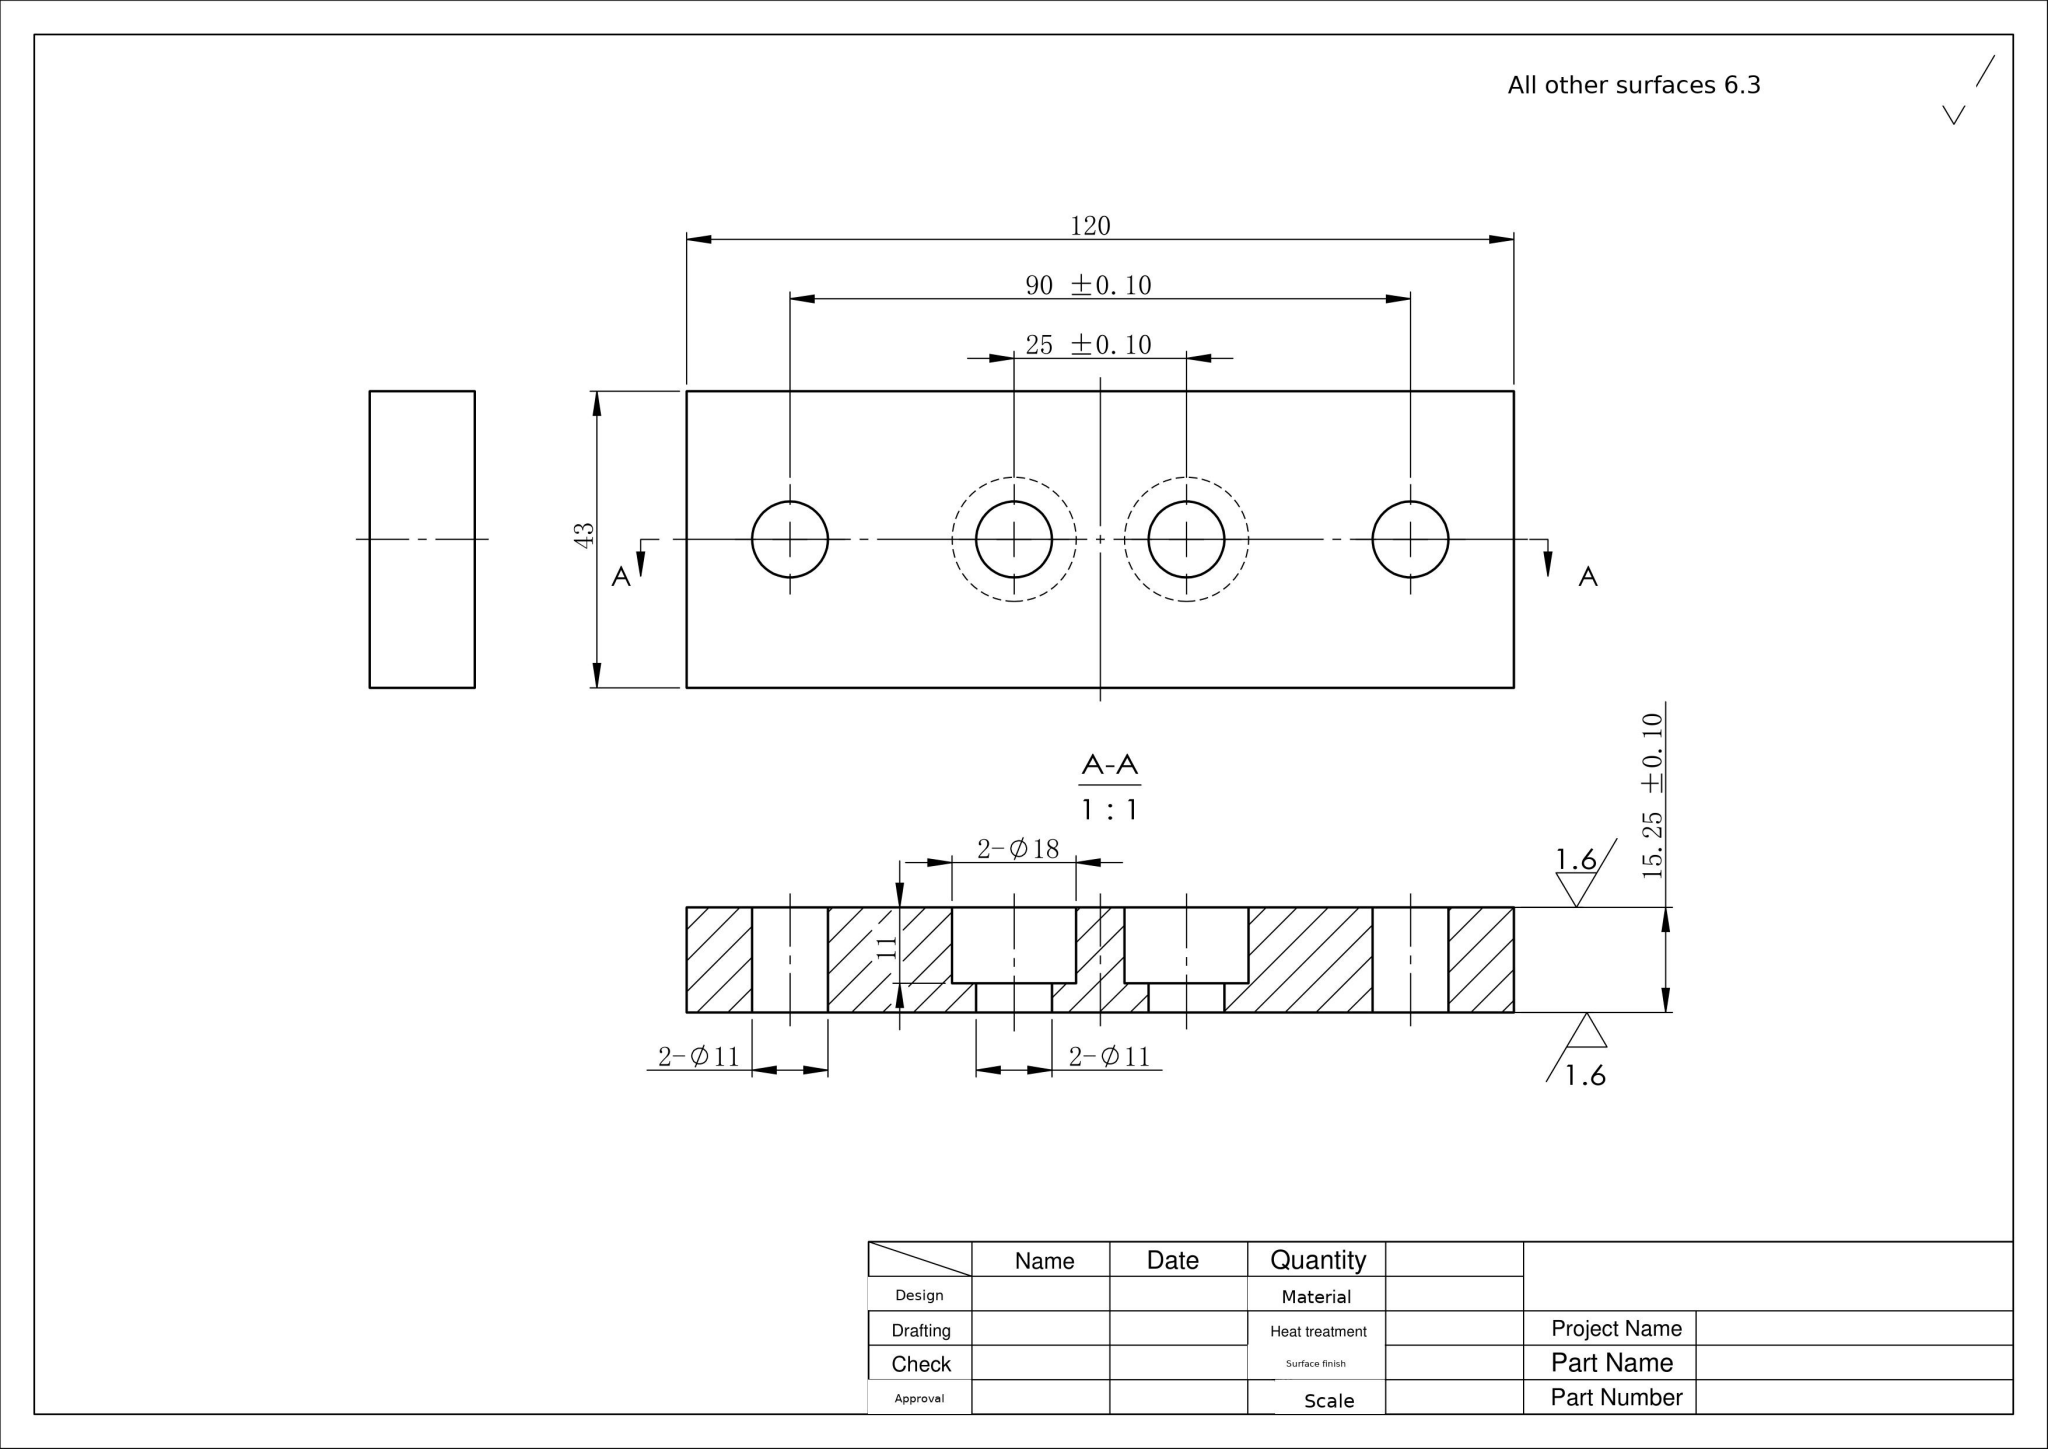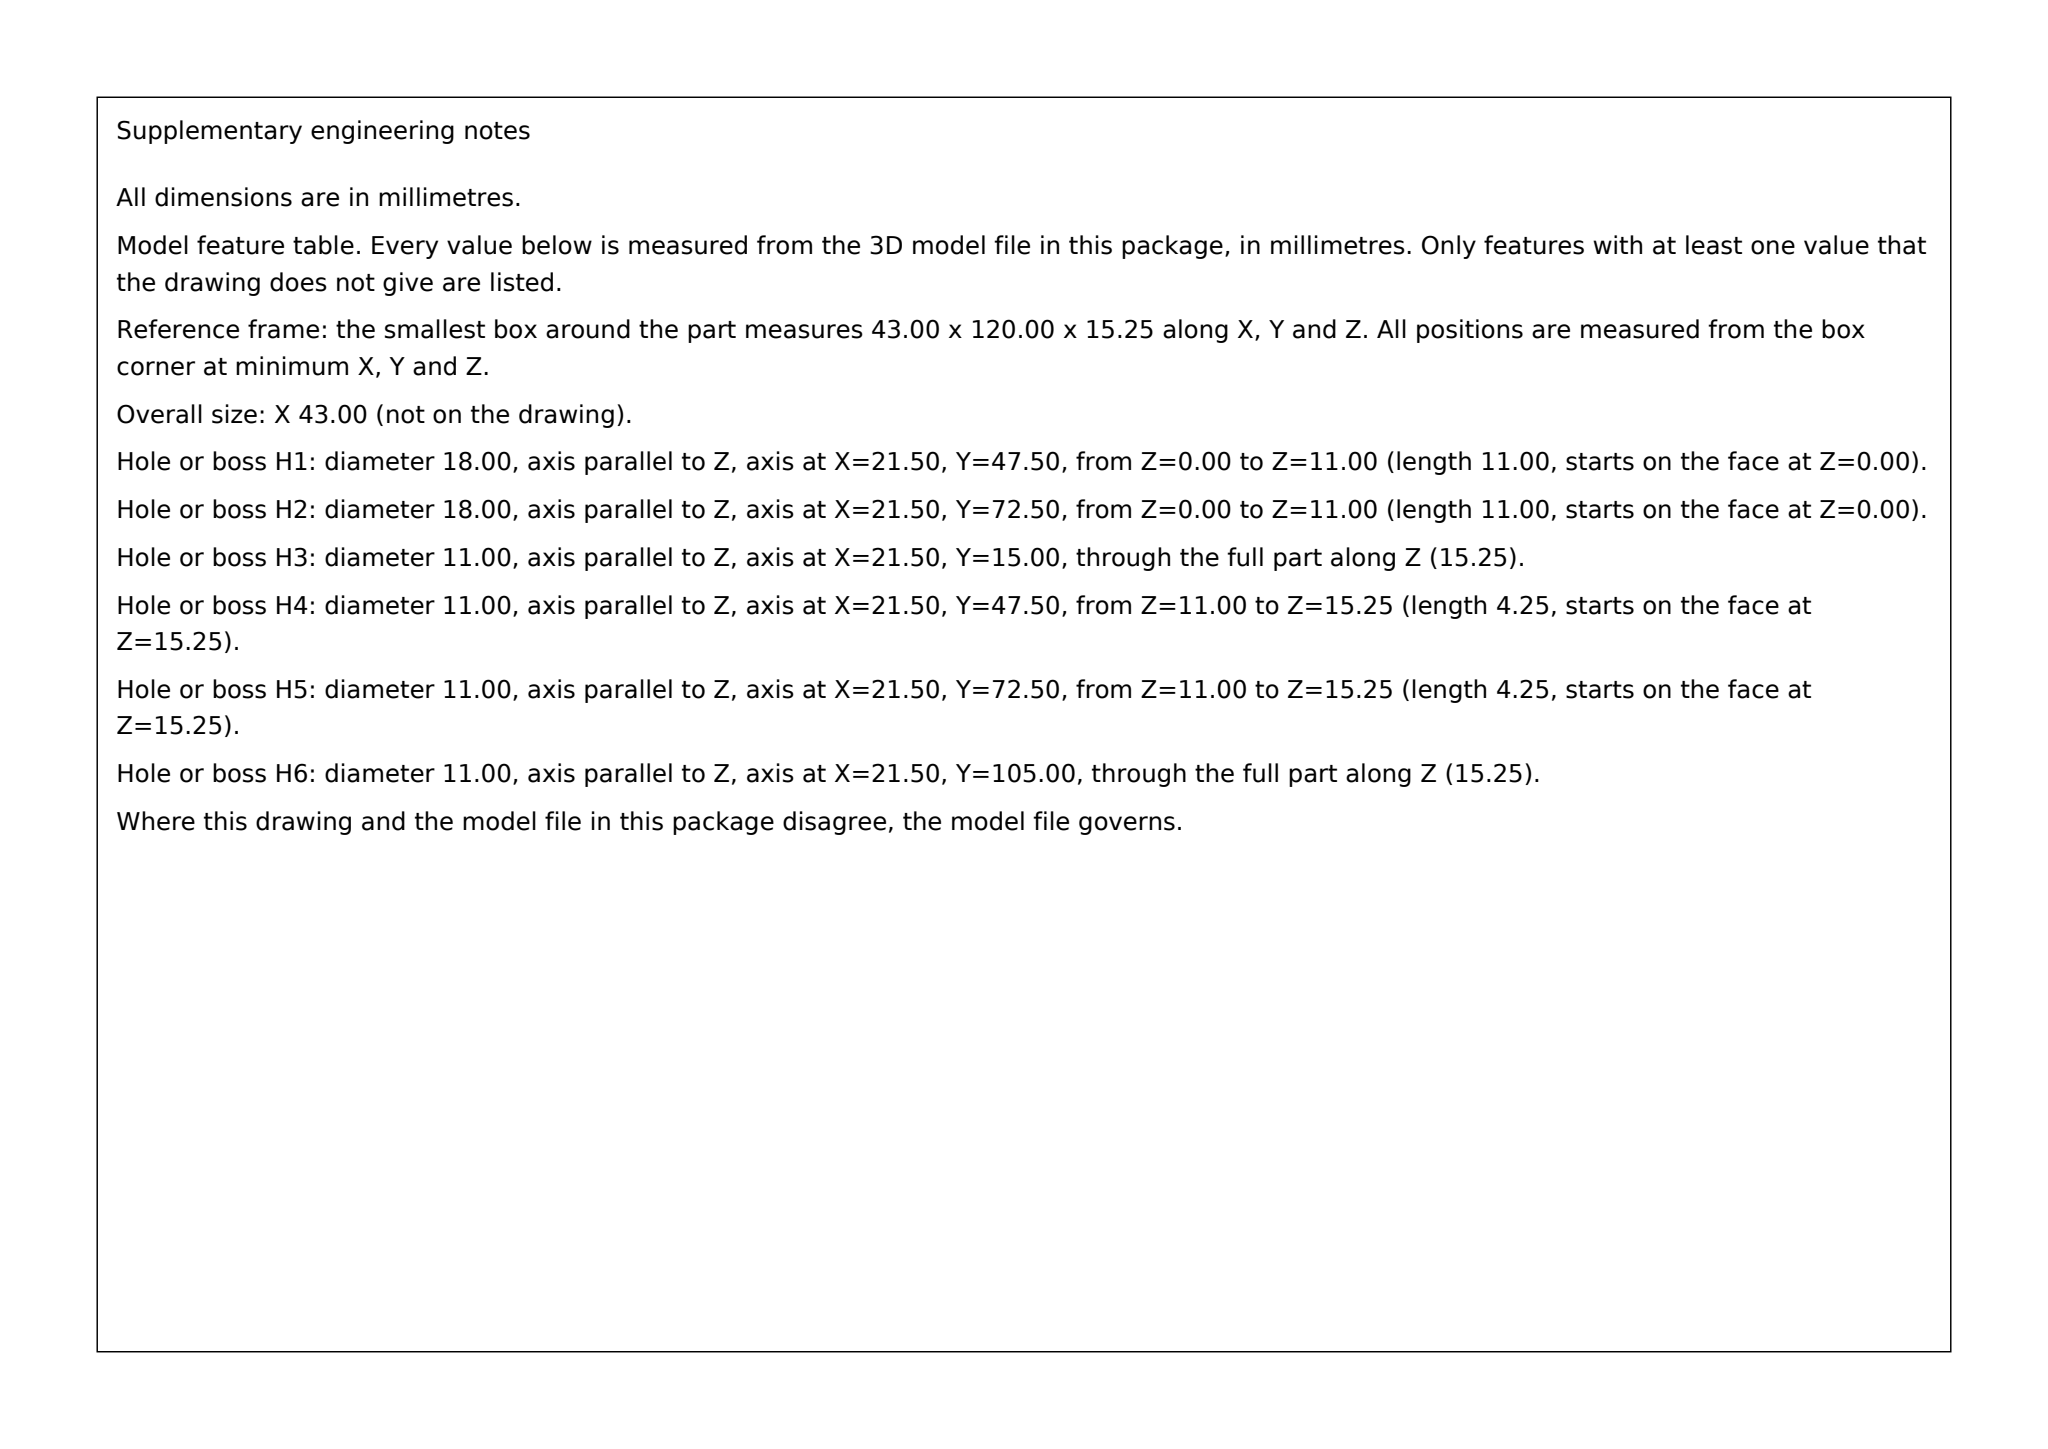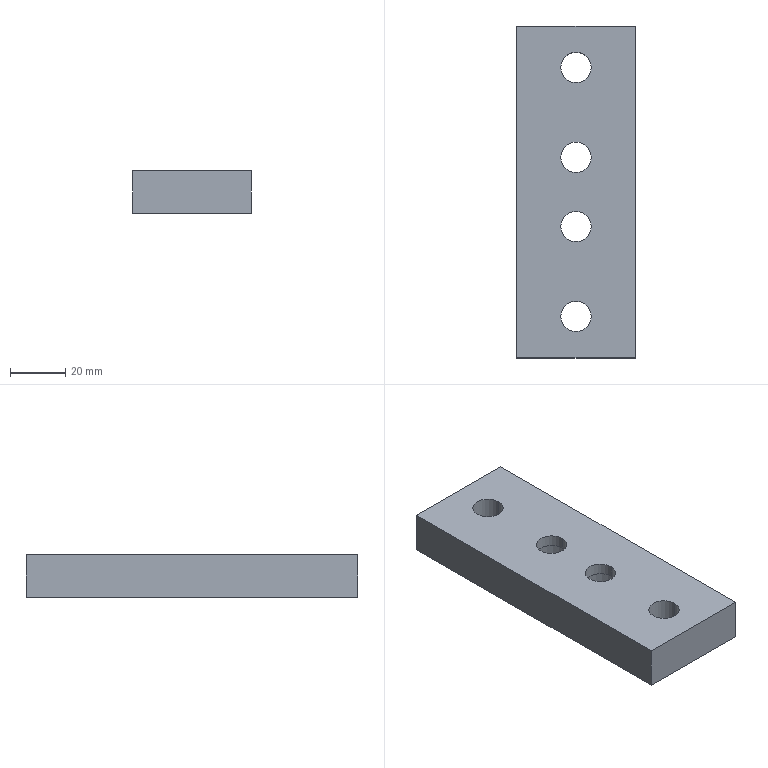Part | SolidWorks | mm | 1 solid | 20 faces | box 43 x 120 x 15.25 mm | volume 69385 mm3 | cylinder 12 | plane 8 | commonest cylinder face diameters 11 x8 18 x4
build123d program:
from build123d import *

# Parameters (mm, degrees)
SKETCH1_W                                        = 43
SKETCH1_H                                        = 120
EXTRUDE1_DEPTH                                   = 15.25
M10_HEX_SOCKET_HEAD_CAP_SCREW_CBORE1_D           = 11
M10_HEX_SOCKET_HEAD_CAP_SCREW_CBORE1_CBORE_D     = 18
M10_HEX_SOCKET_HEAD_CAP_SCREW_CBORE1_CBORE_DEPTH = 11
SKETCH4_R                                        = 5.5
CUT_EXTRUDE1_DEPTH                               = 129.381


with BuildPart() as part:
    # Sketch1 → Extrude1 (new body)
    with BuildSketch(Plane.XY):
        with Locations((21.5, 60)):
            Rectangle(SKETCH1_W, SKETCH1_H)
    extrude(amount=EXTRUDE1_DEPTH)

    # M10 Hex Socket Head Cap Screw CBORE1 (through all)
    with Locations(Plane(origin=(0, 0, 0), x_dir=(-1, 0, 0), z_dir=(0, 0, -1))):
        with Locations((-21.5, 47.5), (-21.5, 72.5)):
            CounterBoreHole(M10_HEX_SOCKET_HEAD_CAP_SCREW_CBORE1_D / 2, M10_HEX_SOCKET_HEAD_CAP_SCREW_CBORE1_CBORE_D / 2, M10_HEX_SOCKET_HEAD_CAP_SCREW_CBORE1_CBORE_DEPTH)

    # Sketch4 → Cut-Extrude1 (cut, through all)
    with BuildSketch(Plane.XY.offset(15.25)):
        with Locations((21.5, 105)):
            Circle(SKETCH4_R)
        with Locations((21.5, 15)):
            Circle(SKETCH4_R)
    extrude(amount=-CUT_EXTRUDE1_DEPTH, mode=Mode.SUBTRACT)


solid = part.part
STEP:
#1=CARTESIAN_POINT('',(16.,15.,0.));
#2=VERTEX_POINT('',#1);
#3=CARTESIAN_POINT('',(27.,15.,0.));
#4=VERTEX_POINT('',#3);
#5=CARTESIAN_POINT('',(21.5,15.,0.));
#6=DIRECTION('',(0.,0.,1.));
#7=DIRECTION('',(1.,0.,0.));
#8=AXIS2_PLACEMENT_3D('',#5,#6,#7);
#9=CIRCLE('',#8,5.5);
#10=EDGE_CURVE('',#2,#4,#9,.T.);
#11=ORIENTED_EDGE('',*,*,#10,.F.);
#12=CARTESIAN_POINT('',(16.,15.,15.25));
#13=VERTEX_POINT('',#12);
#14=CARTESIAN_POINT('',(16.,15.,0.));
#15=DIRECTION('',(0.,0.,1.));
#16=VECTOR('',#15,1000.);
#17=LINE('',#14,#16);
#18=EDGE_CURVE('',#2,#13,#17,.T.);
#19=ORIENTED_EDGE('',*,*,#18,.T.);
#20=CARTESIAN_POINT('',(27.,15.,15.25));
#21=VERTEX_POINT('',#20);
#22=CARTESIAN_POINT('',(21.5,15.,15.25));
#23=DIRECTION('',(0.,0.,1.));
#24=DIRECTION('',(1.,0.,0.));
#25=AXIS2_PLACEMENT_3D('',#22,#23,#24);
#26=CIRCLE('',#25,5.5);
#27=EDGE_CURVE('',#13,#21,#26,.T.);
#28=ORIENTED_EDGE('',*,*,#27,.T.);
#29=CARTESIAN_POINT('',(27.,15.,0.));
#30=DIRECTION('',(0.,0.,1.));
#31=VECTOR('',#30,1000.);
#32=LINE('',#29,#31);
#33=EDGE_CURVE('',#4,#21,#32,.T.);
#34=ORIENTED_EDGE('',*,*,#33,.F.);
#35=EDGE_LOOP('',(#11,#19,#28,#34));
#36=FACE_OUTER_BOUND('',#35,.T.);
#37=CARTESIAN_POINT('',(21.5,15.,0.));
#38=DIRECTION('',(0.,0.,1.));
#39=DIRECTION('',(1.,0.,0.));
#40=AXIS2_PLACEMENT_3D('',#37,#38,#39);
#41=CYLINDRICAL_SURFACE('',#40,5.5);
#42=ADVANCED_FACE('',(#36),#41,.F.);
#43=CARTESIAN_POINT('',(16.,105.,0.));
#44=VERTEX_POINT('',#43);
#45=CARTESIAN_POINT('',(27.,105.,0.));
#46=VERTEX_POINT('',#45);
#47=CARTESIAN_POINT('',(21.5,105.,0.));
#48=DIRECTION('',(0.,0.,1.));
#49=DIRECTION('',(1.,0.,0.));
#50=AXIS2_PLACEMENT_3D('',#47,#48,#49);
#51=CIRCLE('',#50,5.5);
#52=EDGE_CURVE('',#44,#46,#51,.T.);
#53=ORIENTED_EDGE('',*,*,#52,.F.);
#54=CARTESIAN_POINT('',(16.,105.,15.25));
#55=VERTEX_POINT('',#54);
#56=CARTESIAN_POINT('',(16.,105.,0.));
#57=DIRECTION('',(0.,0.,1.));
#58=VECTOR('',#57,1000.);
#59=LINE('',#56,#58);
#60=EDGE_CURVE('',#44,#55,#59,.T.);
#61=ORIENTED_EDGE('',*,*,#60,.T.);
#62=CARTESIAN_POINT('',(27.,105.,15.25));
#63=VERTEX_POINT('',#62);
#64=CARTESIAN_POINT('',(21.5,105.,15.25));
#65=DIRECTION('',(0.,0.,1.));
#66=DIRECTION('',(1.,0.,0.));
#67=AXIS2_PLACEMENT_3D('',#64,#65,#66);
#68=CIRCLE('',#67,5.5);
#69=EDGE_CURVE('',#55,#63,#68,.T.);
#70=ORIENTED_EDGE('',*,*,#69,.T.);
#71=CARTESIAN_POINT('',(27.,105.,0.));
#72=DIRECTION('',(0.,0.,1.));
#73=VECTOR('',#72,1000.);
#74=LINE('',#71,#73);
#75=EDGE_CURVE('',#46,#63,#74,.T.);
#76=ORIENTED_EDGE('',*,*,#75,.F.);
#77=EDGE_LOOP('',(#53,#61,#70,#76));
#78=FACE_OUTER_BOUND('',#77,.T.);
#79=CARTESIAN_POINT('',(21.5,105.,0.));
#80=DIRECTION('',(0.,0.,1.));
#81=DIRECTION('',(1.,0.,0.));
#82=AXIS2_PLACEMENT_3D('',#79,#80,#81);
#83=CYLINDRICAL_SURFACE('',#82,5.5);
#84=ADVANCED_FACE('',(#78),#83,.F.);
#85=CARTESIAN_POINT('',(27.,47.5,15.25));
#86=VERTEX_POINT('',#85);
#87=CARTESIAN_POINT('',(16.,47.5,15.25));
#88=VERTEX_POINT('',#87);
#89=CARTESIAN_POINT('',(21.5,47.5,15.25));
#90=DIRECTION('',(0.,0.,-1.));
#91=DIRECTION('',(-1.,0.,0.));
#92=AXIS2_PLACEMENT_3D('',#89,#90,#91);
#93=CIRCLE('',#92,5.5);
#94=EDGE_CURVE('',#86,#88,#93,.T.);
#95=ORIENTED_EDGE('',*,*,#94,.F.);
#96=CARTESIAN_POINT('',(27.,47.5,11.));
#97=VERTEX_POINT('',#96);
#98=CARTESIAN_POINT('',(27.,47.5,0.));
#99=DIRECTION('',(0.,0.,-1.));
#100=VECTOR('',#99,1000.);
#101=LINE('',#98,#100);
#102=EDGE_CURVE('',#86,#97,#101,.T.);
#103=ORIENTED_EDGE('',*,*,#102,.T.);
#104=CARTESIAN_POINT('',(16.,47.5,11.));
#105=VERTEX_POINT('',#104);
#106=CARTESIAN_POINT('',(21.5,47.5,11.));
#107=DIRECTION('',(0.,0.,-1.));
#108=DIRECTION('',(-1.,0.,0.));
#109=AXIS2_PLACEMENT_3D('',#106,#107,#108);
#110=CIRCLE('',#109,5.5);
#111=EDGE_CURVE('',#97,#105,#110,.T.);
#112=ORIENTED_EDGE('',*,*,#111,.T.);
#113=CARTESIAN_POINT('',(16.,47.5,0.));
#114=DIRECTION('',(0.,0.,-1.));
#115=VECTOR('',#114,1000.);
#116=LINE('',#113,#115);
#117=EDGE_CURVE('',#88,#105,#116,.T.);
#118=ORIENTED_EDGE('',*,*,#117,.F.);
#119=EDGE_LOOP('',(#95,#103,#112,#118));
#120=FACE_OUTER_BOUND('',#119,.T.);
#121=CARTESIAN_POINT('',(21.5,47.5,0.));
#122=DIRECTION('',(0.,0.,-1.));
#123=DIRECTION('',(-1.,0.,0.));
#124=AXIS2_PLACEMENT_3D('',#121,#122,#123);
#125=CYLINDRICAL_SURFACE('',#124,5.5);
#126=ADVANCED_FACE('',(#120),#125,.F.);
#127=CARTESIAN_POINT('',(30.5,47.5,11.));
#128=VERTEX_POINT('',#127);
#129=CARTESIAN_POINT('',(12.5,47.5,11.));
#130=VERTEX_POINT('',#129);
#131=CARTESIAN_POINT('',(21.5,47.5,11.));
#132=DIRECTION('',(0.,0.,-1.));
#133=DIRECTION('',(-1.,0.,0.));
#134=AXIS2_PLACEMENT_3D('',#131,#132,#133);
#135=CIRCLE('',#134,9.);
#136=EDGE_CURVE('',#128,#130,#135,.T.);
#137=ORIENTED_EDGE('',*,*,#136,.F.);
#138=CARTESIAN_POINT('',(30.5,47.5,0.));
#139=VERTEX_POINT('',#138);
#140=CARTESIAN_POINT('',(30.5,47.5,0.));
#141=DIRECTION('',(0.,0.,-1.));
#142=VECTOR('',#141,1000.);
#143=LINE('',#140,#142);
#144=EDGE_CURVE('',#128,#139,#143,.T.);
#145=ORIENTED_EDGE('',*,*,#144,.T.);
#146=CARTESIAN_POINT('',(12.5,47.5,0.));
#147=VERTEX_POINT('',#146);
#148=CARTESIAN_POINT('',(21.5,47.5,0.));
#149=DIRECTION('',(0.,0.,-1.));
#150=DIRECTION('',(-1.,0.,0.));
#151=AXIS2_PLACEMENT_3D('',#148,#149,#150);
#152=CIRCLE('',#151,9.);
#153=EDGE_CURVE('',#139,#147,#152,.T.);
#154=ORIENTED_EDGE('',*,*,#153,.T.);
#155=CARTESIAN_POINT('',(12.5,47.5,0.));
#156=DIRECTION('',(0.,0.,-1.));
#157=VECTOR('',#156,1000.);
#158=LINE('',#155,#157);
#159=EDGE_CURVE('',#130,#147,#158,.T.);
#160=ORIENTED_EDGE('',*,*,#159,.F.);
#161=EDGE_LOOP('',(#137,#145,#154,#160));
#162=FACE_OUTER_BOUND('',#161,.T.);
#163=CARTESIAN_POINT('',(21.5,47.5,0.));
#164=DIRECTION('',(0.,0.,-1.));
#165=DIRECTION('',(-1.,0.,0.));
#166=AXIS2_PLACEMENT_3D('',#163,#164,#165);
#167=CYLINDRICAL_SURFACE('',#166,9.);
#168=ADVANCED_FACE('',(#162),#167,.F.);
#169=CARTESIAN_POINT('',(27.,72.5,15.25));
#170=VERTEX_POINT('',#169);
#171=CARTESIAN_POINT('',(16.,72.5,15.25));
#172=VERTEX_POINT('',#171);
#173=CARTESIAN_POINT('',(21.5,72.5,15.25));
#174=DIRECTION('',(0.,0.,-1.));
#175=DIRECTION('',(-1.,0.,0.));
#176=AXIS2_PLACEMENT_3D('',#173,#174,#175);
#177=CIRCLE('',#176,5.5);
#178=EDGE_CURVE('',#170,#172,#177,.T.);
#179=ORIENTED_EDGE('',*,*,#178,.F.);
#180=CARTESIAN_POINT('',(27.,72.5,11.));
#181=VERTEX_POINT('',#180);
#182=CARTESIAN_POINT('',(27.,72.5,0.));
#183=DIRECTION('',(0.,0.,-1.));
#184=VECTOR('',#183,1000.);
#185=LINE('',#182,#184);
#186=EDGE_CURVE('',#170,#181,#185,.T.);
#187=ORIENTED_EDGE('',*,*,#186,.T.);
#188=CARTESIAN_POINT('',(16.,72.5,11.));
#189=VERTEX_POINT('',#188);
#190=CARTESIAN_POINT('',(21.5,72.5,11.));
#191=DIRECTION('',(0.,0.,-1.));
#192=DIRECTION('',(-1.,0.,0.));
#193=AXIS2_PLACEMENT_3D('',#190,#191,#192);
#194=CIRCLE('',#193,5.5);
#195=EDGE_CURVE('',#181,#189,#194,.T.);
#196=ORIENTED_EDGE('',*,*,#195,.T.);
#197=CARTESIAN_POINT('',(16.,72.5,0.));
#198=DIRECTION('',(0.,0.,-1.));
#199=VECTOR('',#198,1000.);
#200=LINE('',#197,#199);
#201=EDGE_CURVE('',#172,#189,#200,.T.);
#202=ORIENTED_EDGE('',*,*,#201,.F.);
#203=EDGE_LOOP('',(#179,#187,#196,#202));
#204=FACE_OUTER_BOUND('',#203,.T.);
#205=CARTESIAN_POINT('',(21.5,72.5,0.));
#206=DIRECTION('',(0.,0.,-1.));
#207=DIRECTION('',(-1.,0.,0.));
#208=AXIS2_PLACEMENT_3D('',#205,#206,#207);
#209=CYLINDRICAL_SURFACE('',#208,5.5);
#210=ADVANCED_FACE('',(#204),#209,.F.);
#211=CARTESIAN_POINT('',(30.5,72.5,11.));
#212=VERTEX_POINT('',#211);
#213=CARTESIAN_POINT('',(12.5,72.5,11.));
#214=VERTEX_POINT('',#213);
#215=CARTESIAN_POINT('',(21.5,72.5,11.));
#216=DIRECTION('',(0.,0.,-1.));
#217=DIRECTION('',(-1.,0.,0.));
#218=AXIS2_PLACEMENT_3D('',#215,#216,#217);
#219=CIRCLE('',#218,9.);
#220=EDGE_CURVE('',#212,#214,#219,.T.);
#221=ORIENTED_EDGE('',*,*,#220,.F.);
#222=CARTESIAN_POINT('',(30.5,72.5,0.));
#223=VERTEX_POINT('',#222);
#224=CARTESIAN_POINT('',(30.5,72.5,0.));
#225=DIRECTION('',(0.,0.,-1.));
#226=VECTOR('',#225,1000.);
#227=LINE('',#224,#226);
#228=EDGE_CURVE('',#212,#223,#227,.T.);
#229=ORIENTED_EDGE('',*,*,#228,.T.);
#230=CARTESIAN_POINT('',(12.5,72.5,0.));
#231=VERTEX_POINT('',#230);
#232=CARTESIAN_POINT('',(21.5,72.5,0.));
#233=DIRECTION('',(0.,0.,-1.));
#234=DIRECTION('',(-1.,0.,0.));
#235=AXIS2_PLACEMENT_3D('',#232,#233,#234);
#236=CIRCLE('',#235,9.);
#237=EDGE_CURVE('',#223,#231,#236,.T.);
#238=ORIENTED_EDGE('',*,*,#237,.T.);
#239=CARTESIAN_POINT('',(12.5,72.5,0.));
#240=DIRECTION('',(0.,0.,-1.));
#241=VECTOR('',#240,1000.);
#242=LINE('',#239,#241);
#243=EDGE_CURVE('',#214,#231,#242,.T.);
#244=ORIENTED_EDGE('',*,*,#243,.F.);
#245=EDGE_LOOP('',(#221,#229,#238,#244));
#246=FACE_OUTER_BOUND('',#245,.T.);
#247=CARTESIAN_POINT('',(21.5,72.5,0.));
#248=DIRECTION('',(0.,0.,-1.));
#249=DIRECTION('',(-1.,0.,0.));
#250=AXIS2_PLACEMENT_3D('',#247,#248,#249);
#251=CYLINDRICAL_SURFACE('',#250,9.);
#252=ADVANCED_FACE('',(#246),#251,.F.);
#253=CARTESIAN_POINT('',(0.,120.,0.));
#254=VERTEX_POINT('',#253);
#255=CARTESIAN_POINT('',(0.,0.,0.));
#256=VERTEX_POINT('',#255);
#257=CARTESIAN_POINT('',(0.,0.,0.));
#258=DIRECTION('',(0.,-1.,0.));
#259=VECTOR('',#258,1000.);
#260=LINE('',#257,#259);
#261=EDGE_CURVE('',#254,#256,#260,.T.);
#262=ORIENTED_EDGE('',*,*,#261,.T.);
#263=CARTESIAN_POINT('',(0.,0.,15.25));
#264=VERTEX_POINT('',#263);
#265=CARTESIAN_POINT('',(0.,0.,15.25));
#266=DIRECTION('',(0.,0.,-1.));
#267=VECTOR('',#266,1000.);
#268=LINE('',#265,#267);
#269=EDGE_CURVE('',#264,#256,#268,.T.);
#270=ORIENTED_EDGE('',*,*,#269,.F.);
#271=CARTESIAN_POINT('',(0.,120.,15.25));
#272=VERTEX_POINT('',#271);
#273=CARTESIAN_POINT('',(0.,0.,15.25));
#274=DIRECTION('',(0.,-1.,0.));
#275=VECTOR('',#274,1000.);
#276=LINE('',#273,#275);
#277=EDGE_CURVE('',#272,#264,#276,.T.);
#278=ORIENTED_EDGE('',*,*,#277,.F.);
#279=CARTESIAN_POINT('',(0.,120.,15.25));
#280=DIRECTION('',(0.,0.,-1.));
#281=VECTOR('',#280,1000.);
#282=LINE('',#279,#281);
#283=EDGE_CURVE('',#272,#254,#282,.T.);
#284=ORIENTED_EDGE('',*,*,#283,.T.);
#285=EDGE_LOOP('',(#262,#270,#278,#284));
#286=FACE_OUTER_BOUND('',#285,.T.);
#287=CARTESIAN_POINT('',(0.,0.,15.25));
#288=DIRECTION('',(1.,0.,0.));
#289=DIRECTION('',(0.,0.,-1.));
#290=AXIS2_PLACEMENT_3D('',#287,#288,#289);
#291=PLANE('',#290);
#292=ADVANCED_FACE('',(#286),#291,.F.);
#293=CARTESIAN_POINT('',(43.,0.,0.));
#294=VERTEX_POINT('',#293);
#295=CARTESIAN_POINT('',(0.,0.,0.));
#296=DIRECTION('',(1.,0.,0.));
#297=VECTOR('',#296,1000.);
#298=LINE('',#295,#297);
#299=EDGE_CURVE('',#256,#294,#298,.T.);
#300=ORIENTED_EDGE('',*,*,#299,.T.);
#301=CARTESIAN_POINT('',(43.,0.,15.25));
#302=VERTEX_POINT('',#301);
#303=CARTESIAN_POINT('',(43.,0.,15.25));
#304=DIRECTION('',(0.,0.,-1.));
#305=VECTOR('',#304,1000.);
#306=LINE('',#303,#305);
#307=EDGE_CURVE('',#302,#294,#306,.T.);
#308=ORIENTED_EDGE('',*,*,#307,.F.);
#309=CARTESIAN_POINT('',(0.,0.,15.25));
#310=DIRECTION('',(1.,0.,0.));
#311=VECTOR('',#310,1000.);
#312=LINE('',#309,#311);
#313=EDGE_CURVE('',#264,#302,#312,.T.);
#314=ORIENTED_EDGE('',*,*,#313,.F.);
#315=ORIENTED_EDGE('',*,*,#269,.T.);
#316=EDGE_LOOP('',(#300,#308,#314,#315));
#317=FACE_OUTER_BOUND('',#316,.T.);
#318=CARTESIAN_POINT('',(0.,0.,15.25));
#319=DIRECTION('',(0.,1.,0.));
#320=DIRECTION('',(0.,0.,1.));
#321=AXIS2_PLACEMENT_3D('',#318,#319,#320);
#322=PLANE('',#321);
#323=ADVANCED_FACE('',(#317),#322,.F.);
#324=CARTESIAN_POINT('',(43.,120.,0.));
#325=VERTEX_POINT('',#324);
#326=CARTESIAN_POINT('',(43.,0.,0.));
#327=DIRECTION('',(0.,1.,0.));
#328=VECTOR('',#327,1000.);
#329=LINE('',#326,#328);
#330=EDGE_CURVE('',#294,#325,#329,.T.);
#331=ORIENTED_EDGE('',*,*,#330,.T.);
#332=CARTESIAN_POINT('',(43.,120.,15.25));
#333=VERTEX_POINT('',#332);
#334=CARTESIAN_POINT('',(43.,120.,15.25));
#335=DIRECTION('',(0.,0.,-1.));
#336=VECTOR('',#335,1000.);
#337=LINE('',#334,#336);
#338=EDGE_CURVE('',#333,#325,#337,.T.);
#339=ORIENTED_EDGE('',*,*,#338,.F.);
#340=CARTESIAN_POINT('',(43.,0.,15.25));
#341=DIRECTION('',(0.,1.,0.));
#342=VECTOR('',#341,1000.);
#343=LINE('',#340,#342);
#344=EDGE_CURVE('',#302,#333,#343,.T.);
#345=ORIENTED_EDGE('',*,*,#344,.F.);
#346=ORIENTED_EDGE('',*,*,#307,.T.);
#347=EDGE_LOOP('',(#331,#339,#345,#346));
#348=FACE_OUTER_BOUND('',#347,.T.);
#349=CARTESIAN_POINT('',(43.,0.,15.25));
#350=DIRECTION('',(-1.,0.,0.));
#351=DIRECTION('',(0.,0.,1.));
#352=AXIS2_PLACEMENT_3D('',#349,#350,#351);
#353=PLANE('',#352);
#354=ADVANCED_FACE('',(#348),#353,.F.);
#355=CARTESIAN_POINT('',(0.,120.,0.));
#356=DIRECTION('',(-1.,0.,0.));
#357=VECTOR('',#356,1000.);
#358=LINE('',#355,#357);
#359=EDGE_CURVE('',#325,#254,#358,.T.);
#360=ORIENTED_EDGE('',*,*,#359,.T.);
#361=ORIENTED_EDGE('',*,*,#283,.F.);
#362=CARTESIAN_POINT('',(0.,120.,15.25));
#363=DIRECTION('',(-1.,0.,0.));
#364=VECTOR('',#363,1000.);
#365=LINE('',#362,#364);
#366=EDGE_CURVE('',#333,#272,#365,.T.);
#367=ORIENTED_EDGE('',*,*,#366,.F.);
#368=ORIENTED_EDGE('',*,*,#338,.T.);
#369=EDGE_LOOP('',(#360,#361,#367,#368));
#370=FACE_OUTER_BOUND('',#369,.T.);
#371=CARTESIAN_POINT('',(0.,120.,15.25));
#372=DIRECTION('',(0.,-1.,0.));
#373=DIRECTION('',(0.,0.,-1.));
#374=AXIS2_PLACEMENT_3D('',#371,#372,#373);
#375=PLANE('',#374);
#376=ADVANCED_FACE('',(#370),#375,.F.);
#377=CARTESIAN_POINT('',(21.5,15.,15.25));
#378=DIRECTION('',(0.,0.,1.));
#379=DIRECTION('',(1.,0.,0.));
#380=AXIS2_PLACEMENT_3D('',#377,#378,#379);
#381=CIRCLE('',#380,5.5);
#382=EDGE_CURVE('',#21,#13,#381,.T.);
#383=ORIENTED_EDGE('',*,*,#382,.F.);
#384=ORIENTED_EDGE('',*,*,#27,.F.);
#385=EDGE_LOOP('',(#383,#384));
#386=FACE_BOUND('',#385,.T.);
#387=CARTESIAN_POINT('',(21.5,105.,15.25));
#388=DIRECTION('',(0.,0.,1.));
#389=DIRECTION('',(1.,0.,0.));
#390=AXIS2_PLACEMENT_3D('',#387,#388,#389);
#391=CIRCLE('',#390,5.5);
#392=EDGE_CURVE('',#63,#55,#391,.T.);
#393=ORIENTED_EDGE('',*,*,#392,.F.);
#394=ORIENTED_EDGE('',*,*,#69,.F.);
#395=EDGE_LOOP('',(#393,#394));
#396=FACE_BOUND('',#395,.T.);
#397=CARTESIAN_POINT('',(21.5,47.5,15.25));
#398=DIRECTION('',(0.,0.,-1.));
#399=DIRECTION('',(-1.,0.,0.));
#400=AXIS2_PLACEMENT_3D('',#397,#398,#399);
#401=CIRCLE('',#400,5.5);
#402=EDGE_CURVE('',#88,#86,#401,.T.);
#403=ORIENTED_EDGE('',*,*,#402,.T.);
#404=ORIENTED_EDGE('',*,*,#94,.T.);
#405=EDGE_LOOP('',(#403,#404));
#406=FACE_BOUND('',#405,.T.);
#407=CARTESIAN_POINT('',(21.5,72.5,15.25));
#408=DIRECTION('',(0.,0.,-1.));
#409=DIRECTION('',(-1.,0.,0.));
#410=AXIS2_PLACEMENT_3D('',#407,#408,#409);
#411=CIRCLE('',#410,5.5);
#412=EDGE_CURVE('',#172,#170,#411,.T.);
#413=ORIENTED_EDGE('',*,*,#412,.T.);
#414=ORIENTED_EDGE('',*,*,#178,.T.);
#415=EDGE_LOOP('',(#413,#414));
#416=FACE_BOUND('',#415,.T.);
#417=ORIENTED_EDGE('',*,*,#277,.T.);
#418=ORIENTED_EDGE('',*,*,#313,.T.);
#419=ORIENTED_EDGE('',*,*,#344,.T.);
#420=ORIENTED_EDGE('',*,*,#366,.T.);
#421=EDGE_LOOP('',(#417,#418,#419,#420));
#422=FACE_OUTER_BOUND('',#421,.T.);
#423=CARTESIAN_POINT('',(0.,120.,15.25));
#424=DIRECTION('',(0.,0.,-1.));
#425=DIRECTION('',(-1.,0.,0.));
#426=AXIS2_PLACEMENT_3D('',#423,#424,#425);
#427=PLANE('',#426);
#428=ADVANCED_FACE('',(#386,#396,#406,#416,#422),#427,.F.);
#429=CARTESIAN_POINT('',(21.5,15.,0.));
#430=DIRECTION('',(0.,0.,1.));
#431=DIRECTION('',(1.,0.,0.));
#432=AXIS2_PLACEMENT_3D('',#429,#430,#431);
#433=CIRCLE('',#432,5.5);
#434=EDGE_CURVE('',#4,#2,#433,.T.);
#435=ORIENTED_EDGE('',*,*,#434,.T.);
#436=ORIENTED_EDGE('',*,*,#10,.T.);
#437=EDGE_LOOP('',(#435,#436));
#438=FACE_BOUND('',#437,.T.);
#439=CARTESIAN_POINT('',(21.5,105.,0.));
#440=DIRECTION('',(0.,0.,1.));
#441=DIRECTION('',(1.,0.,0.));
#442=AXIS2_PLACEMENT_3D('',#439,#440,#441);
#443=CIRCLE('',#442,5.5);
#444=EDGE_CURVE('',#46,#44,#443,.T.);
#445=ORIENTED_EDGE('',*,*,#444,.T.);
#446=ORIENTED_EDGE('',*,*,#52,.T.);
#447=EDGE_LOOP('',(#445,#446));
#448=FACE_BOUND('',#447,.T.);
#449=CARTESIAN_POINT('',(21.5,47.5,0.));
#450=DIRECTION('',(0.,0.,-1.));
#451=DIRECTION('',(-1.,0.,0.));
#452=AXIS2_PLACEMENT_3D('',#449,#450,#451);
#453=CIRCLE('',#452,9.);
#454=EDGE_CURVE('',#147,#139,#453,.T.);
#455=ORIENTED_EDGE('',*,*,#454,.F.);
#456=ORIENTED_EDGE('',*,*,#153,.F.);
#457=EDGE_LOOP('',(#455,#456));
#458=FACE_BOUND('',#457,.T.);
#459=CARTESIAN_POINT('',(21.5,72.5,0.));
#460=DIRECTION('',(0.,0.,-1.));
#461=DIRECTION('',(-1.,0.,0.));
#462=AXIS2_PLACEMENT_3D('',#459,#460,#461);
#463=CIRCLE('',#462,9.);
#464=EDGE_CURVE('',#231,#223,#463,.T.);
#465=ORIENTED_EDGE('',*,*,#464,.F.);
#466=ORIENTED_EDGE('',*,*,#237,.F.);
#467=EDGE_LOOP('',(#465,#466));
#468=FACE_BOUND('',#467,.T.);
#469=ORIENTED_EDGE('',*,*,#261,.F.);
#470=ORIENTED_EDGE('',*,*,#359,.F.);
#471=ORIENTED_EDGE('',*,*,#330,.F.);
#472=ORIENTED_EDGE('',*,*,#299,.F.);
#473=EDGE_LOOP('',(#469,#470,#471,#472));
#474=FACE_OUTER_BOUND('',#473,.T.);
#475=CARTESIAN_POINT('',(0.,120.,0.));
#476=DIRECTION('',(0.,0.,-1.));
#477=DIRECTION('',(-1.,0.,0.));
#478=AXIS2_PLACEMENT_3D('',#475,#476,#477);
#479=PLANE('',#478);
#480=ADVANCED_FACE('',(#438,#448,#458,#468,#474),#479,.T.);
#481=ORIENTED_EDGE('',*,*,#228,.F.);
#482=CARTESIAN_POINT('',(21.5,72.5,11.));
#483=DIRECTION('',(0.,0.,-1.));
#484=DIRECTION('',(-1.,0.,0.));
#485=AXIS2_PLACEMENT_3D('',#482,#483,#484);
#486=CIRCLE('',#485,9.);
#487=EDGE_CURVE('',#214,#212,#486,.T.);
#488=ORIENTED_EDGE('',*,*,#487,.F.);
#489=ORIENTED_EDGE('',*,*,#243,.T.);
#490=ORIENTED_EDGE('',*,*,#464,.T.);
#491=EDGE_LOOP('',(#481,#488,#489,#490));
#492=FACE_OUTER_BOUND('',#491,.T.);
#493=CARTESIAN_POINT('',(21.5,72.5,0.));
#494=DIRECTION('',(0.,0.,-1.));
#495=DIRECTION('',(-1.,0.,0.));
#496=AXIS2_PLACEMENT_3D('',#493,#494,#495);
#497=CYLINDRICAL_SURFACE('',#496,9.);
#498=ADVANCED_FACE('',(#492),#497,.F.);
#499=CARTESIAN_POINT('',(21.5,72.5,11.));
#500=DIRECTION('',(0.,0.,-1.));
#501=DIRECTION('',(-1.,0.,0.));
#502=AXIS2_PLACEMENT_3D('',#499,#500,#501);
#503=CIRCLE('',#502,5.5);
#504=EDGE_CURVE('',#189,#181,#503,.T.);
#505=ORIENTED_EDGE('',*,*,#504,.F.);
#506=ORIENTED_EDGE('',*,*,#195,.F.);
#507=EDGE_LOOP('',(#505,#506));
#508=FACE_BOUND('',#507,.T.);
#509=ORIENTED_EDGE('',*,*,#487,.T.);
#510=ORIENTED_EDGE('',*,*,#220,.T.);
#511=EDGE_LOOP('',(#509,#510));
#512=FACE_OUTER_BOUND('',#511,.T.);
#513=CARTESIAN_POINT('',(27.,72.5,11.));
#514=DIRECTION('',(0.,0.,1.));
#515=DIRECTION('',(1.,0.,0.));
#516=AXIS2_PLACEMENT_3D('',#513,#514,#515);
#517=PLANE('',#516);
#518=ADVANCED_FACE('',(#508,#512),#517,.F.);
#519=ORIENTED_EDGE('',*,*,#186,.F.);
#520=ORIENTED_EDGE('',*,*,#412,.F.);
#521=ORIENTED_EDGE('',*,*,#201,.T.);
#522=ORIENTED_EDGE('',*,*,#504,.T.);
#523=EDGE_LOOP('',(#519,#520,#521,#522));
#524=FACE_OUTER_BOUND('',#523,.T.);
#525=CARTESIAN_POINT('',(21.5,72.5,0.));
#526=DIRECTION('',(0.,0.,-1.));
#527=DIRECTION('',(-1.,0.,0.));
#528=AXIS2_PLACEMENT_3D('',#525,#526,#527);
#529=CYLINDRICAL_SURFACE('',#528,5.5);
#530=ADVANCED_FACE('',(#524),#529,.F.);
#531=ORIENTED_EDGE('',*,*,#144,.F.);
#532=CARTESIAN_POINT('',(21.5,47.5,11.));
#533=DIRECTION('',(0.,0.,-1.));
#534=DIRECTION('',(-1.,0.,0.));
#535=AXIS2_PLACEMENT_3D('',#532,#533,#534);
#536=CIRCLE('',#535,9.);
#537=EDGE_CURVE('',#130,#128,#536,.T.);
#538=ORIENTED_EDGE('',*,*,#537,.F.);
#539=ORIENTED_EDGE('',*,*,#159,.T.);
#540=ORIENTED_EDGE('',*,*,#454,.T.);
#541=EDGE_LOOP('',(#531,#538,#539,#540));
#542=FACE_OUTER_BOUND('',#541,.T.);
#543=CARTESIAN_POINT('',(21.5,47.5,0.));
#544=DIRECTION('',(0.,0.,-1.));
#545=DIRECTION('',(-1.,0.,0.));
#546=AXIS2_PLACEMENT_3D('',#543,#544,#545);
#547=CYLINDRICAL_SURFACE('',#546,9.);
#548=ADVANCED_FACE('',(#542),#547,.F.);
#549=CARTESIAN_POINT('',(21.5,47.5,11.));
#550=DIRECTION('',(0.,0.,-1.));
#551=DIRECTION('',(-1.,0.,0.));
#552=AXIS2_PLACEMENT_3D('',#549,#550,#551);
#553=CIRCLE('',#552,5.5);
#554=EDGE_CURVE('',#105,#97,#553,.T.);
#555=ORIENTED_EDGE('',*,*,#554,.F.);
#556=ORIENTED_EDGE('',*,*,#111,.F.);
#557=EDGE_LOOP('',(#555,#556));
#558=FACE_BOUND('',#557,.T.);
#559=ORIENTED_EDGE('',*,*,#537,.T.);
#560=ORIENTED_EDGE('',*,*,#136,.T.);
#561=EDGE_LOOP('',(#559,#560));
#562=FACE_OUTER_BOUND('',#561,.T.);
#563=CARTESIAN_POINT('',(27.,47.5,11.));
#564=DIRECTION('',(0.,0.,1.));
#565=DIRECTION('',(1.,0.,0.));
#566=AXIS2_PLACEMENT_3D('',#563,#564,#565);
#567=PLANE('',#566);
#568=ADVANCED_FACE('',(#558,#562),#567,.F.);
#569=ORIENTED_EDGE('',*,*,#102,.F.);
#570=ORIENTED_EDGE('',*,*,#402,.F.);
#571=ORIENTED_EDGE('',*,*,#117,.T.);
#572=ORIENTED_EDGE('',*,*,#554,.T.);
#573=EDGE_LOOP('',(#569,#570,#571,#572));
#574=FACE_OUTER_BOUND('',#573,.T.);
#575=CARTESIAN_POINT('',(21.5,47.5,0.));
#576=DIRECTION('',(0.,0.,-1.));
#577=DIRECTION('',(-1.,0.,0.));
#578=AXIS2_PLACEMENT_3D('',#575,#576,#577);
#579=CYLINDRICAL_SURFACE('',#578,5.5);
#580=ADVANCED_FACE('',(#574),#579,.F.);
#581=ORIENTED_EDGE('',*,*,#60,.F.);
#582=ORIENTED_EDGE('',*,*,#444,.F.);
#583=ORIENTED_EDGE('',*,*,#75,.T.);
#584=ORIENTED_EDGE('',*,*,#392,.T.);
#585=EDGE_LOOP('',(#581,#582,#583,#584));
#586=FACE_OUTER_BOUND('',#585,.T.);
#587=CARTESIAN_POINT('',(21.5,105.,0.));
#588=DIRECTION('',(0.,0.,1.));
#589=DIRECTION('',(1.,0.,0.));
#590=AXIS2_PLACEMENT_3D('',#587,#588,#589);
#591=CYLINDRICAL_SURFACE('',#590,5.5);
#592=ADVANCED_FACE('',(#586),#591,.F.);
#593=ORIENTED_EDGE('',*,*,#18,.F.);
#594=ORIENTED_EDGE('',*,*,#434,.F.);
#595=ORIENTED_EDGE('',*,*,#33,.T.);
#596=ORIENTED_EDGE('',*,*,#382,.T.);
#597=EDGE_LOOP('',(#593,#594,#595,#596));
#598=FACE_OUTER_BOUND('',#597,.T.);
#599=CARTESIAN_POINT('',(21.5,15.,0.));
#600=DIRECTION('',(0.,0.,1.));
#601=DIRECTION('',(1.,0.,0.));
#602=AXIS2_PLACEMENT_3D('',#599,#600,#601);
#603=CYLINDRICAL_SURFACE('',#602,5.5);
#604=ADVANCED_FACE('',(#598),#603,.F.);
#605=CLOSED_SHELL('',(#42,#84,#126,#168,#210,#252,#292,#323,#354,#376,#428,#480,#498,#518,#530,#548,#568,#580,#592,#604));
#606=MANIFOLD_SOLID_BREP('',#605);
#607=CARTESIAN_POINT('',(0.,0.,0.));
#608=DIRECTION('',(0.,0.,1.));
#609=DIRECTION('',(1.,0.,0.));
#610=AXIS2_PLACEMENT_3D('',#607,#608,#609);
#611=(LENGTH_UNIT()NAMED_UNIT(*)SI_UNIT(.MILLI.,.METRE.));
#612=UNCERTAINTY_MEASURE_WITH_UNIT(LENGTH_MEASURE(0.00001),#611,'','');
#613=(NAMED_UNIT(*)PLANE_ANGLE_UNIT()SI_UNIT($,.RADIAN.));
#614=(NAMED_UNIT(*)SI_UNIT($,.STERADIAN.)SOLID_ANGLE_UNIT());
#615=(GEOMETRIC_REPRESENTATION_CONTEXT(3)GLOBAL_UNCERTAINTY_ASSIGNED_CONTEXT((#612))GLOBAL_UNIT_ASSIGNED_CONTEXT((#611,#613,#614))REPRESENTATION_CONTEXT('',''));
#616=ADVANCED_BREP_SHAPE_REPRESENTATION('',(#606,#610),#615);